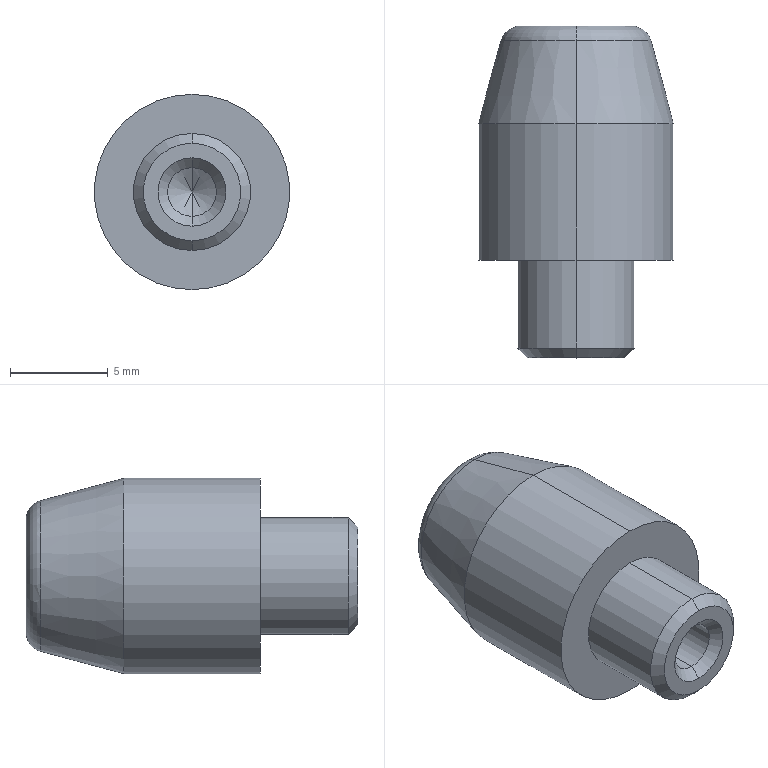Component | SolidWorks | MA060.03.03-02-1 | 1 solid | 19 faces | box 10 x 17 x 10 mm | volume 944 mm3 | cone 8 | cylinder 6 | plane 3 | torus 2 | commonest cylinder face diameters 2.5 x2 6 x2 10 x2 | material 45#
build123d program:
from build123d import *

# Parameters (mm, degrees)
M3_TAPPED_HOLE1_D     = 2.5
M3_TAPPED_HOLE1_DEPTH = 7.5
M3_TAPPED_HOLE1_TIP   = 0.7511
CHAMFER1_SIZE         = 0.5
CHAMFER2_SIZE         = 5
CHAMFER2_SIZE2        = 1.34
FILLET1_R             = 1


with BuildPart() as part:
    # Sketch1 → Revolve1 (revolve)
    with BuildSketch(Plane.XY, mode=Mode.PRIVATE) as revolve1_sk:
        Polygon((0, 0), (0, 17), (5, 17), (5, 5), (3, 5), (3, 0), align=None)
    revolve(revolve1_sk.sketch.rotate(Axis((0, 0, 0), (0, 1, 0)), 90), axis=Axis((0, 0, 0), (0, 1, 0)))

    # M3 Tapped Hole1
    with Locations(Plane(origin=(0, 0, 0), x_dir=(0, 0, -1), z_dir=(0, -1, 0))):
        with Locations((0, 0)):
            Hole(M3_TAPPED_HOLE1_D / 2, depth=M3_TAPPED_HOLE1_DEPTH)
            with Locations((0, 0, -(M3_TAPPED_HOLE1_DEPTH + M3_TAPPED_HOLE1_TIP / 2))):  # 118° drill point
                Cone(0, M3_TAPPED_HOLE1_D / 2, M3_TAPPED_HOLE1_TIP, mode=Mode.SUBTRACT)

    # Chamfer1
    chamfer1_edges = [part.edges().sort_by_distance(p)[0] for p in [
        (0, 0, -1.25),
        (0, 0, 3),
    ]]
    chamfer(chamfer1_edges, length=CHAMFER1_SIZE)

    # Chamfer2
    chamfer2_edges = [part.edges().sort_by_distance(p)[0] for p in [
        (0, 17, 5),
    ]]
    chamfer2_side = [part.faces().sort_by_distance(p)[0] for p in [
        (0, 11, 5),
    ]]
    chamfer(chamfer2_edges, length=CHAMFER2_SIZE, length2=CHAMFER2_SIZE2, reference=chamfer2_side[0])

    # Fillet1
    fillet1_edges = [part.edges().sort_by_distance(p)[0] for p in [
        (0, 17, 3.66),
    ]]
    fillet(fillet1_edges, radius=FILLET1_R)


solid = part.part

# Placed as in the assembly
solid = solid.moved(Location((-41, 73.053, 0), (0, 0, 0)))
STEP:
#1=CARTESIAN_POINT('',(-1.614,3.516,-0.1519));
#2=VERTEX_POINT('',#1);
#3=CARTESIAN_POINT('',(-1.614,3.516,0.1519));
#4=VERTEX_POINT('',#3);
#5=CARTESIAN_POINT('',(-1.614,3.516,-0.));
#6=DIRECTION('',(0.,-1.,0.));
#7=DIRECTION('',(0.,0.,1.));
#8=AXIS2_PLACEMENT_3D('',#5,#6,#7);
#9=CIRCLE('',#8,0.1519);
#10=EDGE_CURVE('',#2,#4,#9,.T.);
#11=ORIENTED_EDGE('',*,*,#10,.F.);
#12=CARTESIAN_POINT('',(-1.614,3.545,-0.1139));
#13=VERTEX_POINT('',#12);
#14=CARTESIAN_POINT('',(-1.614,3.506,-0.1139));
#15=DIRECTION('',(1.,0.,0.));
#16=DIRECTION('',(0.,0.,-1.));
#17=AXIS2_PLACEMENT_3D('',#14,#15,#16);
#18=CIRCLE('',#17,0.03937);
#19=EDGE_CURVE('',#2,#13,#18,.T.);
#20=ORIENTED_EDGE('',*,*,#19,.T.);
#21=CARTESIAN_POINT('',(-1.614,3.545,0.1139));
#22=VERTEX_POINT('',#21);
#23=CARTESIAN_POINT('',(-1.614,3.545,-0.));
#24=DIRECTION('',(0.,1.,0.));
#25=DIRECTION('',(0.,0.,1.));
#26=AXIS2_PLACEMENT_3D('',#23,#24,#25);
#27=CIRCLE('',#26,0.1139);
#28=EDGE_CURVE('',#22,#13,#27,.T.);
#29=ORIENTED_EDGE('',*,*,#28,.F.);
#30=CARTESIAN_POINT('',(-1.614,3.506,0.1139));
#31=DIRECTION('',(-1.,0.,0.));
#32=DIRECTION('',(0.,0.,1.));
#33=AXIS2_PLACEMENT_3D('',#30,#31,#32);
#34=CIRCLE('',#33,0.03937);
#35=EDGE_CURVE('',#4,#22,#34,.T.);
#36=ORIENTED_EDGE('',*,*,#35,.F.);
#37=EDGE_LOOP('',(#11,#20,#29,#36));
#38=FACE_OUTER_BOUND('',#37,.T.);
#39=CARTESIAN_POINT('',(-1.614,3.506,-0.));
#40=DIRECTION('',(0.,1.,0.));
#41=DIRECTION('',(0.,0.,1.));
#42=AXIS2_PLACEMENT_3D('',#39,#40,#41);
#43=TOROIDAL_SURFACE('',#42,0.1139,0.03937);
#44=ADVANCED_FACE('',(#38),#43,.T.);
#45=ORIENTED_EDGE('',*,*,#10,.T.);
#46=CARTESIAN_POINT('',(-1.614,3.349,0.1969));
#47=VERTEX_POINT('',#46);
#48=CARTESIAN_POINT('',(-1.614,3.349,0.1969));
#49=DIRECTION('',(0.,-0.9659,0.2588));
#50=VECTOR('',#49,39.37);
#51=LINE('',#48,#50);
#52=EDGE_CURVE('',#4,#47,#51,.T.);
#53=ORIENTED_EDGE('',*,*,#52,.T.);
#54=CARTESIAN_POINT('',(-1.614,3.349,-0.1969));
#55=VERTEX_POINT('',#54);
#56=CARTESIAN_POINT('',(-1.614,3.349,-0.));
#57=DIRECTION('',(0.,-1.,0.));
#58=DIRECTION('',(0.,0.,1.));
#59=AXIS2_PLACEMENT_3D('',#56,#57,#58);
#60=CIRCLE('',#59,0.1969);
#61=EDGE_CURVE('',#55,#47,#60,.T.);
#62=ORIENTED_EDGE('',*,*,#61,.F.);
#63=CARTESIAN_POINT('',(-1.614,3.349,-0.1969));
#64=DIRECTION('',(0.,-0.9659,-0.2588));
#65=VECTOR('',#64,39.37);
#66=LINE('',#63,#65);
#67=EDGE_CURVE('',#2,#55,#66,.T.);
#68=ORIENTED_EDGE('',*,*,#67,.F.);
#69=EDGE_LOOP('',(#45,#53,#62,#68));
#70=FACE_OUTER_BOUND('',#69,.T.);
#71=CARTESIAN_POINT('',(-1.614,3.349,-0.));
#72=DIRECTION('',(0.,-1.,0.));
#73=DIRECTION('',(0.,0.,-1.));
#74=AXIS2_PLACEMENT_3D('',#71,#72,#73);
#75=CONICAL_SURFACE('',#74,0.1969,0.2618);
#76=ADVANCED_FACE('',(#70),#75,.T.);
#77=CARTESIAN_POINT('',(-1.614,2.896,0.04921));
#78=VERTEX_POINT('',#77);
#79=CARTESIAN_POINT('',(-1.614,2.896,-0.04921));
#80=VERTEX_POINT('',#79);
#81=CARTESIAN_POINT('',(-1.614,2.896,-0.));
#82=DIRECTION('',(0.,-1.,0.));
#83=DIRECTION('',(0.,0.,-1.));
#84=AXIS2_PLACEMENT_3D('',#81,#82,#83);
#85=CIRCLE('',#84,0.04921);
#86=EDGE_CURVE('',#78,#80,#85,.T.);
#87=ORIENTED_EDGE('',*,*,#86,.F.);
#88=CARTESIAN_POINT('',(-1.614,2.876,0.0689));
#89=VERTEX_POINT('',#88);
#90=CARTESIAN_POINT('',(-1.614,2.896,0.04921));
#91=DIRECTION('',(0.,-0.7071,0.7071));
#92=VECTOR('',#91,39.37);
#93=LINE('',#90,#92);
#94=EDGE_CURVE('',#78,#89,#93,.T.);
#95=ORIENTED_EDGE('',*,*,#94,.T.);
#96=CARTESIAN_POINT('',(-1.614,2.876,-0.0689));
#97=VERTEX_POINT('',#96);
#98=CARTESIAN_POINT('',(-1.614,2.876,-0.));
#99=DIRECTION('',(0.,1.,0.));
#100=DIRECTION('',(0.,0.,-1.));
#101=AXIS2_PLACEMENT_3D('',#98,#99,#100);
#102=CIRCLE('',#101,0.0689);
#103=EDGE_CURVE('',#97,#89,#102,.T.);
#104=ORIENTED_EDGE('',*,*,#103,.F.);
#105=CARTESIAN_POINT('',(-1.614,2.896,-0.04921));
#106=DIRECTION('',(0.,-0.7071,-0.7071));
#107=VECTOR('',#106,39.37);
#108=LINE('',#105,#107);
#109=EDGE_CURVE('',#80,#97,#108,.T.);
#110=ORIENTED_EDGE('',*,*,#109,.F.);
#111=EDGE_LOOP('',(#87,#95,#104,#110));
#112=FACE_OUTER_BOUND('',#111,.T.);
#113=CARTESIAN_POINT('',(-1.614,2.896,-0.));
#114=DIRECTION('',(0.,-1.,0.));
#115=DIRECTION('',(0.,0.,-1.));
#116=AXIS2_PLACEMENT_3D('',#113,#114,#115);
#117=CONICAL_SURFACE('',#116,0.04921,0.7854);
#118=ADVANCED_FACE('',(#112),#117,.F.);
#119=CARTESIAN_POINT('',(-1.614,2.876,-0.09843));
#120=VERTEX_POINT('',#119);
#121=CARTESIAN_POINT('',(-1.614,2.876,0.09843));
#122=VERTEX_POINT('',#121);
#123=CARTESIAN_POINT('',(-1.614,2.876,-0.));
#124=DIRECTION('',(0.,-1.,0.));
#125=DIRECTION('',(0.,0.,-1.));
#126=AXIS2_PLACEMENT_3D('',#123,#124,#125);
#127=CIRCLE('',#126,0.09843);
#128=EDGE_CURVE('',#120,#122,#127,.T.);
#129=ORIENTED_EDGE('',*,*,#128,.F.);
#130=CARTESIAN_POINT('',(-1.614,2.896,-0.1181));
#131=VERTEX_POINT('',#130);
#132=CARTESIAN_POINT('',(-1.614,2.876,-0.09843));
#133=DIRECTION('',(0.,0.7071,-0.7071));
#134=VECTOR('',#133,39.37);
#135=LINE('',#132,#134);
#136=EDGE_CURVE('',#120,#131,#135,.T.);
#137=ORIENTED_EDGE('',*,*,#136,.T.);
#138=CARTESIAN_POINT('',(-1.614,2.896,0.1181));
#139=VERTEX_POINT('',#138);
#140=CARTESIAN_POINT('',(-1.614,2.896,-0.));
#141=DIRECTION('',(0.,1.,0.));
#142=DIRECTION('',(0.,0.,-1.));
#143=AXIS2_PLACEMENT_3D('',#140,#141,#142);
#144=CIRCLE('',#143,0.1181);
#145=EDGE_CURVE('',#139,#131,#144,.T.);
#146=ORIENTED_EDGE('',*,*,#145,.F.);
#147=CARTESIAN_POINT('',(-1.614,2.876,0.09843));
#148=DIRECTION('',(0.,0.7071,0.7071));
#149=VECTOR('',#148,39.37);
#150=LINE('',#147,#149);
#151=EDGE_CURVE('',#122,#139,#150,.T.);
#152=ORIENTED_EDGE('',*,*,#151,.F.);
#153=EDGE_LOOP('',(#129,#137,#146,#152));
#154=FACE_OUTER_BOUND('',#153,.T.);
#155=CARTESIAN_POINT('',(-1.614,2.876,-0.));
#156=DIRECTION('',(0.,1.,0.));
#157=DIRECTION('',(0.,0.,1.));
#158=AXIS2_PLACEMENT_3D('',#155,#156,#157);
#159=CONICAL_SURFACE('',#158,0.09843,0.7854);
#160=ADVANCED_FACE('',(#154),#159,.T.);
#161=CARTESIAN_POINT('',(-1.614,3.171,0.04921));
#162=VERTEX_POINT('',#161);
#163=CARTESIAN_POINT('',(-1.614,3.171,-0.04921));
#164=VERTEX_POINT('',#163);
#165=CARTESIAN_POINT('',(-1.614,3.171,-0.));
#166=DIRECTION('',(0.,-1.,0.));
#167=DIRECTION('',(0.,0.,-1.));
#168=AXIS2_PLACEMENT_3D('',#165,#166,#167);
#169=CIRCLE('',#168,0.04921);
#170=EDGE_CURVE('',#162,#164,#169,.T.);
#171=ORIENTED_EDGE('',*,*,#170,.F.);
#172=CARTESIAN_POINT('',(-1.614,2.876,0.04921));
#173=DIRECTION('',(0.,-1.,0.));
#174=VECTOR('',#173,39.37);
#175=LINE('',#172,#174);
#176=EDGE_CURVE('',#162,#78,#175,.T.);
#177=ORIENTED_EDGE('',*,*,#176,.T.);
#178=ORIENTED_EDGE('',*,*,#86,.T.);
#179=CARTESIAN_POINT('',(-1.614,2.876,-0.04921));
#180=DIRECTION('',(0.,-1.,0.));
#181=VECTOR('',#180,39.37);
#182=LINE('',#179,#181);
#183=EDGE_CURVE('',#164,#80,#182,.T.);
#184=ORIENTED_EDGE('',*,*,#183,.F.);
#185=EDGE_LOOP('',(#171,#177,#178,#184));
#186=FACE_OUTER_BOUND('',#185,.T.);
#187=CARTESIAN_POINT('',(-1.614,2.876,-0.));
#188=DIRECTION('',(0.,-1.,0.));
#189=DIRECTION('',(0.,0.,-1.));
#190=AXIS2_PLACEMENT_3D('',#187,#188,#189);
#191=CYLINDRICAL_SURFACE('',#190,0.04921);
#192=ADVANCED_FACE('',(#186),#191,.F.);
#193=CARTESIAN_POINT('',(-1.614,3.201,-0.));
#194=VERTEX_POINT('',#193);
#195=CARTESIAN_POINT('',(-1.614,3.171,-0.04921));
#196=DIRECTION('',(0.,-0.515,-0.8572));
#197=VECTOR('',#196,39.37);
#198=LINE('',#195,#197);
#199=EDGE_CURVE('',#194,#164,#198,.T.);
#200=ORIENTED_EDGE('',*,*,#199,.F.);
#201=CARTESIAN_POINT('',(-1.614,3.171,0.04921));
#202=DIRECTION('',(0.,-0.515,0.8572));
#203=VECTOR('',#202,39.37);
#204=LINE('',#201,#203);
#205=EDGE_CURVE('',#194,#162,#204,.T.);
#206=ORIENTED_EDGE('',*,*,#205,.T.);
#207=ORIENTED_EDGE('',*,*,#170,.T.);
#208=EDGE_LOOP('',(#200,#206,#207));
#209=FACE_OUTER_BOUND('',#208,.T.);
#210=CARTESIAN_POINT('',(-1.614,3.171,-0.));
#211=DIRECTION('',(0.,-1.,0.));
#212=DIRECTION('',(0.,0.,-1.));
#213=AXIS2_PLACEMENT_3D('',#210,#211,#212);
#214=CONICAL_SURFACE('',#213,0.04921,1.03);
#215=ADVANCED_FACE('',(#209),#214,.F.);
#216=CARTESIAN_POINT('',(-1.614,3.073,-0.1181));
#217=VERTEX_POINT('',#216);
#218=CARTESIAN_POINT('',(-1.614,3.073,0.1181));
#219=VERTEX_POINT('',#218);
#220=CARTESIAN_POINT('',(-1.614,3.073,-0.));
#221=DIRECTION('',(0.,-1.,0.));
#222=DIRECTION('',(0.,0.,-1.));
#223=AXIS2_PLACEMENT_3D('',#220,#221,#222);
#224=CIRCLE('',#223,0.1181);
#225=EDGE_CURVE('',#217,#219,#224,.T.);
#226=ORIENTED_EDGE('',*,*,#225,.T.);
#227=CARTESIAN_POINT('',(-1.614,2.876,0.1181));
#228=DIRECTION('',(0.,-1.,0.));
#229=VECTOR('',#228,39.37);
#230=LINE('',#227,#229);
#231=EDGE_CURVE('',#219,#139,#230,.T.);
#232=ORIENTED_EDGE('',*,*,#231,.T.);
#233=ORIENTED_EDGE('',*,*,#145,.T.);
#234=CARTESIAN_POINT('',(-1.614,2.876,-0.1181));
#235=DIRECTION('',(0.,-1.,0.));
#236=VECTOR('',#235,39.37);
#237=LINE('',#234,#236);
#238=EDGE_CURVE('',#217,#131,#237,.T.);
#239=ORIENTED_EDGE('',*,*,#238,.F.);
#240=EDGE_LOOP('',(#226,#232,#233,#239));
#241=FACE_OUTER_BOUND('',#240,.T.);
#242=CARTESIAN_POINT('',(-1.614,2.876,-0.));
#243=DIRECTION('',(0.,-1.,0.));
#244=DIRECTION('',(0.,0.,-1.));
#245=AXIS2_PLACEMENT_3D('',#242,#243,#244);
#246=CYLINDRICAL_SURFACE('',#245,0.1181);
#247=ADVANCED_FACE('',(#241),#246,.T.);
#248=ORIENTED_EDGE('',*,*,#61,.T.);
#249=CARTESIAN_POINT('',(-1.614,3.073,0.1969));
#250=VERTEX_POINT('',#249);
#251=CARTESIAN_POINT('',(-1.614,2.876,0.1969));
#252=DIRECTION('',(0.,-1.,0.));
#253=VECTOR('',#252,39.37);
#254=LINE('',#251,#253);
#255=EDGE_CURVE('',#47,#250,#254,.T.);
#256=ORIENTED_EDGE('',*,*,#255,.T.);
#257=CARTESIAN_POINT('',(-1.614,3.073,-0.1969));
#258=VERTEX_POINT('',#257);
#259=CARTESIAN_POINT('',(-1.614,3.073,-0.));
#260=DIRECTION('',(0.,-1.,0.));
#261=DIRECTION('',(0.,0.,-1.));
#262=AXIS2_PLACEMENT_3D('',#259,#260,#261);
#263=CIRCLE('',#262,0.1969);
#264=EDGE_CURVE('',#258,#250,#263,.T.);
#265=ORIENTED_EDGE('',*,*,#264,.F.);
#266=CARTESIAN_POINT('',(-1.614,2.876,-0.1969));
#267=DIRECTION('',(0.,-1.,0.));
#268=VECTOR('',#267,39.37);
#269=LINE('',#266,#268);
#270=EDGE_CURVE('',#55,#258,#269,.T.);
#271=ORIENTED_EDGE('',*,*,#270,.F.);
#272=EDGE_LOOP('',(#248,#256,#265,#271));
#273=FACE_OUTER_BOUND('',#272,.T.);
#274=CARTESIAN_POINT('',(-1.614,2.876,-0.));
#275=DIRECTION('',(0.,-1.,0.));
#276=DIRECTION('',(0.,0.,-1.));
#277=AXIS2_PLACEMENT_3D('',#274,#275,#276);
#278=CYLINDRICAL_SURFACE('',#277,0.1969);
#279=ADVANCED_FACE('',(#273),#278,.T.);
#280=CARTESIAN_POINT('',(-1.614,2.876,-0.));
#281=DIRECTION('',(0.,-1.,0.));
#282=DIRECTION('',(0.,0.,-1.));
#283=AXIS2_PLACEMENT_3D('',#280,#281,#282);
#284=CIRCLE('',#283,0.09843);
#285=EDGE_CURVE('',#122,#120,#284,.T.);
#286=ORIENTED_EDGE('',*,*,#285,.T.);
#287=ORIENTED_EDGE('',*,*,#128,.T.);
#288=EDGE_LOOP('',(#286,#287));
#289=FACE_OUTER_BOUND('',#288,.T.);
#290=ORIENTED_EDGE('',*,*,#103,.T.);
#291=CARTESIAN_POINT('',(-1.614,2.876,-0.));
#292=DIRECTION('',(0.,1.,0.));
#293=DIRECTION('',(0.,0.,-1.));
#294=AXIS2_PLACEMENT_3D('',#291,#292,#293);
#295=CIRCLE('',#294,0.0689);
#296=EDGE_CURVE('',#89,#97,#295,.T.);
#297=ORIENTED_EDGE('',*,*,#296,.T.);
#298=EDGE_LOOP('',(#290,#297));
#299=FACE_BOUND('',#298,.T.);
#300=CARTESIAN_POINT('',(-1.496,2.876,-0.));
#301=DIRECTION('',(0.,-1.,0.));
#302=DIRECTION('',(0.,0.,-1.));
#303=AXIS2_PLACEMENT_3D('',#300,#301,#302);
#304=PLANE('',#303);
#305=ADVANCED_FACE('',(#289,#299),#304,.T.);
#306=ORIENTED_EDGE('',*,*,#28,.T.);
#307=CARTESIAN_POINT('',(-1.614,3.545,-0.));
#308=DIRECTION('',(0.,1.,0.));
#309=DIRECTION('',(0.,0.,1.));
#310=AXIS2_PLACEMENT_3D('',#307,#308,#309);
#311=CIRCLE('',#310,0.1139);
#312=EDGE_CURVE('',#13,#22,#311,.T.);
#313=ORIENTED_EDGE('',*,*,#312,.T.);
#314=EDGE_LOOP('',(#306,#313));
#315=FACE_OUTER_BOUND('',#314,.T.);
#316=CARTESIAN_POINT('',(-1.614,3.545,-0.));
#317=DIRECTION('',(0.,1.,0.));
#318=DIRECTION('',(0.,0.,1.));
#319=AXIS2_PLACEMENT_3D('',#316,#317,#318);
#320=PLANE('',#319);
#321=ADVANCED_FACE('',(#315),#320,.T.);
#322=ORIENTED_EDGE('',*,*,#255,.F.);
#323=CARTESIAN_POINT('',(-1.614,3.349,-0.));
#324=DIRECTION('',(0.,-1.,0.));
#325=DIRECTION('',(0.,0.,1.));
#326=AXIS2_PLACEMENT_3D('',#323,#324,#325);
#327=CIRCLE('',#326,0.1969);
#328=EDGE_CURVE('',#47,#55,#327,.T.);
#329=ORIENTED_EDGE('',*,*,#328,.T.);
#330=ORIENTED_EDGE('',*,*,#270,.T.);
#331=CARTESIAN_POINT('',(-1.614,3.073,-0.));
#332=DIRECTION('',(0.,-1.,0.));
#333=DIRECTION('',(0.,0.,-1.));
#334=AXIS2_PLACEMENT_3D('',#331,#332,#333);
#335=CIRCLE('',#334,0.1969);
#336=EDGE_CURVE('',#250,#258,#335,.T.);
#337=ORIENTED_EDGE('',*,*,#336,.F.);
#338=EDGE_LOOP('',(#322,#329,#330,#337));
#339=FACE_OUTER_BOUND('',#338,.T.);
#340=CARTESIAN_POINT('',(-1.614,2.876,-0.));
#341=DIRECTION('',(0.,-1.,0.));
#342=DIRECTION('',(0.,0.,-1.));
#343=AXIS2_PLACEMENT_3D('',#340,#341,#342);
#344=CYLINDRICAL_SURFACE('',#343,0.1969);
#345=ADVANCED_FACE('',(#339),#344,.T.);
#346=ORIENTED_EDGE('',*,*,#264,.T.);
#347=ORIENTED_EDGE('',*,*,#336,.T.);
#348=EDGE_LOOP('',(#346,#347));
#349=FACE_OUTER_BOUND('',#348,.T.);
#350=ORIENTED_EDGE('',*,*,#225,.F.);
#351=CARTESIAN_POINT('',(-1.614,3.073,-0.));
#352=DIRECTION('',(0.,-1.,0.));
#353=DIRECTION('',(0.,0.,-1.));
#354=AXIS2_PLACEMENT_3D('',#351,#352,#353);
#355=CIRCLE('',#354,0.1181);
#356=EDGE_CURVE('',#219,#217,#355,.T.);
#357=ORIENTED_EDGE('',*,*,#356,.F.);
#358=EDGE_LOOP('',(#350,#357));
#359=FACE_BOUND('',#358,.T.);
#360=CARTESIAN_POINT('',(-1.417,3.073,-0.));
#361=DIRECTION('',(0.,-1.,0.));
#362=DIRECTION('',(0.,0.,-1.));
#363=AXIS2_PLACEMENT_3D('',#360,#361,#362);
#364=PLANE('',#363);
#365=ADVANCED_FACE('',(#349,#359),#364,.T.);
#366=ORIENTED_EDGE('',*,*,#231,.F.);
#367=ORIENTED_EDGE('',*,*,#356,.T.);
#368=ORIENTED_EDGE('',*,*,#238,.T.);
#369=CARTESIAN_POINT('',(-1.614,2.896,-0.));
#370=DIRECTION('',(0.,1.,0.));
#371=DIRECTION('',(0.,0.,-1.));
#372=AXIS2_PLACEMENT_3D('',#369,#370,#371);
#373=CIRCLE('',#372,0.1181);
#374=EDGE_CURVE('',#131,#139,#373,.T.);
#375=ORIENTED_EDGE('',*,*,#374,.T.);
#376=EDGE_LOOP('',(#366,#367,#368,#375));
#377=FACE_OUTER_BOUND('',#376,.T.);
#378=CARTESIAN_POINT('',(-1.614,2.876,-0.));
#379=DIRECTION('',(0.,-1.,0.));
#380=DIRECTION('',(0.,0.,-1.));
#381=AXIS2_PLACEMENT_3D('',#378,#379,#380);
#382=CYLINDRICAL_SURFACE('',#381,0.1181);
#383=ADVANCED_FACE('',(#377),#382,.T.);
#384=ORIENTED_EDGE('',*,*,#205,.F.);
#385=ORIENTED_EDGE('',*,*,#199,.T.);
#386=CARTESIAN_POINT('',(-1.614,3.171,-0.));
#387=DIRECTION('',(0.,-1.,0.));
#388=DIRECTION('',(0.,0.,-1.));
#389=AXIS2_PLACEMENT_3D('',#386,#387,#388);
#390=CIRCLE('',#389,0.04921);
#391=EDGE_CURVE('',#164,#162,#390,.T.);
#392=ORIENTED_EDGE('',*,*,#391,.T.);
#393=EDGE_LOOP('',(#384,#385,#392));
#394=FACE_OUTER_BOUND('',#393,.T.);
#395=CARTESIAN_POINT('',(-1.614,3.171,-0.));
#396=DIRECTION('',(0.,-1.,0.));
#397=DIRECTION('',(0.,0.,-1.));
#398=AXIS2_PLACEMENT_3D('',#395,#396,#397);
#399=CONICAL_SURFACE('',#398,0.04921,1.03);
#400=ADVANCED_FACE('',(#394),#399,.F.);
#401=ORIENTED_EDGE('',*,*,#176,.F.);
#402=ORIENTED_EDGE('',*,*,#391,.F.);
#403=ORIENTED_EDGE('',*,*,#183,.T.);
#404=CARTESIAN_POINT('',(-1.614,2.896,-0.));
#405=DIRECTION('',(0.,-1.,0.));
#406=DIRECTION('',(0.,0.,-1.));
#407=AXIS2_PLACEMENT_3D('',#404,#405,#406);
#408=CIRCLE('',#407,0.04921);
#409=EDGE_CURVE('',#80,#78,#408,.T.);
#410=ORIENTED_EDGE('',*,*,#409,.T.);
#411=EDGE_LOOP('',(#401,#402,#403,#410));
#412=FACE_OUTER_BOUND('',#411,.T.);
#413=CARTESIAN_POINT('',(-1.614,2.876,-0.));
#414=DIRECTION('',(0.,-1.,0.));
#415=DIRECTION('',(0.,0.,-1.));
#416=AXIS2_PLACEMENT_3D('',#413,#414,#415);
#417=CYLINDRICAL_SURFACE('',#416,0.04921);
#418=ADVANCED_FACE('',(#412),#417,.F.);
#419=ORIENTED_EDGE('',*,*,#136,.F.);
#420=ORIENTED_EDGE('',*,*,#285,.F.);
#421=ORIENTED_EDGE('',*,*,#151,.T.);
#422=ORIENTED_EDGE('',*,*,#374,.F.);
#423=EDGE_LOOP('',(#419,#420,#421,#422));
#424=FACE_OUTER_BOUND('',#423,.T.);
#425=CARTESIAN_POINT('',(-1.614,2.876,-0.));
#426=DIRECTION('',(0.,1.,0.));
#427=DIRECTION('',(0.,0.,1.));
#428=AXIS2_PLACEMENT_3D('',#425,#426,#427);
#429=CONICAL_SURFACE('',#428,0.09843,0.7854);
#430=ADVANCED_FACE('',(#424),#429,.T.);
#431=ORIENTED_EDGE('',*,*,#94,.F.);
#432=ORIENTED_EDGE('',*,*,#409,.F.);
#433=ORIENTED_EDGE('',*,*,#109,.T.);
#434=ORIENTED_EDGE('',*,*,#296,.F.);
#435=EDGE_LOOP('',(#431,#432,#433,#434));
#436=FACE_OUTER_BOUND('',#435,.T.);
#437=CARTESIAN_POINT('',(-1.614,2.896,-0.));
#438=DIRECTION('',(0.,-1.,0.));
#439=DIRECTION('',(0.,0.,-1.));
#440=AXIS2_PLACEMENT_3D('',#437,#438,#439);
#441=CONICAL_SURFACE('',#440,0.04921,0.7854);
#442=ADVANCED_FACE('',(#436),#441,.F.);
#443=ORIENTED_EDGE('',*,*,#52,.F.);
#444=CARTESIAN_POINT('',(-1.614,3.516,-0.));
#445=DIRECTION('',(0.,-1.,0.));
#446=DIRECTION('',(0.,0.,1.));
#447=AXIS2_PLACEMENT_3D('',#444,#445,#446);
#448=CIRCLE('',#447,0.1519);
#449=EDGE_CURVE('',#4,#2,#448,.T.);
#450=ORIENTED_EDGE('',*,*,#449,.T.);
#451=ORIENTED_EDGE('',*,*,#67,.T.);
#452=ORIENTED_EDGE('',*,*,#328,.F.);
#453=EDGE_LOOP('',(#443,#450,#451,#452));
#454=FACE_OUTER_BOUND('',#453,.T.);
#455=CARTESIAN_POINT('',(-1.614,3.349,-0.));
#456=DIRECTION('',(0.,-1.,0.));
#457=DIRECTION('',(0.,0.,-1.));
#458=AXIS2_PLACEMENT_3D('',#455,#456,#457);
#459=CONICAL_SURFACE('',#458,0.1969,0.2618);
#460=ADVANCED_FACE('',(#454),#459,.T.);
#461=ORIENTED_EDGE('',*,*,#19,.F.);
#462=ORIENTED_EDGE('',*,*,#449,.F.);
#463=ORIENTED_EDGE('',*,*,#35,.T.);
#464=ORIENTED_EDGE('',*,*,#312,.F.);
#465=EDGE_LOOP('',(#461,#462,#463,#464));
#466=FACE_OUTER_BOUND('',#465,.T.);
#467=CARTESIAN_POINT('',(-1.614,3.506,-0.));
#468=DIRECTION('',(0.,1.,0.));
#469=DIRECTION('',(0.,0.,1.));
#470=AXIS2_PLACEMENT_3D('',#467,#468,#469);
#471=TOROIDAL_SURFACE('',#470,0.1139,0.03937);
#472=ADVANCED_FACE('',(#466),#471,.T.);
#473=CLOSED_SHELL('',(#44,#76,#118,#160,#192,#215,#247,#279,#305,#321,#345,#365,#383,#400,#418,#430,#442,#460,#472));
#474=MANIFOLD_SOLID_BREP('',#473);
#475=CARTESIAN_POINT('',(0.,0.,0.));
#476=DIRECTION('',(0.,0.,1.));
#477=DIRECTION('',(1.,0.,0.));
#478=AXIS2_PLACEMENT_3D('',#475,#476,#477);
#479=(LENGTH_UNIT()NAMED_UNIT(*)SI_UNIT($,.METRE.));
#480=LENGTH_MEASURE_WITH_UNIT(LENGTH_MEASURE(0.0254),#479);
#481=DIMENSIONAL_EXPONENTS(1.,0.,0.,0.,0.,0.,0.);
#482=(CONVERSION_BASED_UNIT('',#480)LENGTH_UNIT()NAMED_UNIT(#481));
#483=UNCERTAINTY_MEASURE_WITH_UNIT(LENGTH_MEASURE(0.00001),#482,'','');
#484=(NAMED_UNIT(*)PLANE_ANGLE_UNIT()SI_UNIT($,.RADIAN.));
#485=(NAMED_UNIT(*)SI_UNIT($,.STERADIAN.)SOLID_ANGLE_UNIT());
#486=(GEOMETRIC_REPRESENTATION_CONTEXT(3)GLOBAL_UNCERTAINTY_ASSIGNED_CONTEXT((#483))GLOBAL_UNIT_ASSIGNED_CONTEXT((#482,#484,#485))REPRESENTATION_CONTEXT('',''));
#487=ADVANCED_BREP_SHAPE_REPRESENTATION('',(#474,#478),#486);
#488=COLOUR_RGB('',0.7922,0.8196,0.9333);
#489=FILL_AREA_STYLE_COLOUR('',#488);
#490=FILL_AREA_STYLE('',(#489));
#491=SURFACE_STYLE_FILL_AREA(#490);
#492=SURFACE_SIDE_STYLE('',(#491));
#493=SURFACE_STYLE_USAGE(.BOTH.,#492);
#494=PRESENTATION_STYLE_ASSIGNMENT((#493));
#495=STYLED_ITEM('',(#494),#474);
#496=(LENGTH_UNIT()NAMED_UNIT(*)SI_UNIT($,.METRE.));
#497=LENGTH_MEASURE_WITH_UNIT(LENGTH_MEASURE(0.0254),#496);
#498=DIMENSIONAL_EXPONENTS(1.,0.,0.,0.,0.,0.,0.);
#499=(CONVERSION_BASED_UNIT('',#497)LENGTH_UNIT()NAMED_UNIT(#498));
#500=UNCERTAINTY_MEASURE_WITH_UNIT(LENGTH_MEASURE(0.00001),#499,'','');
#501=(NAMED_UNIT(*)PLANE_ANGLE_UNIT()SI_UNIT($,.RADIAN.));
#502=(NAMED_UNIT(*)SI_UNIT($,.STERADIAN.)SOLID_ANGLE_UNIT());
#503=(GEOMETRIC_REPRESENTATION_CONTEXT(3)GLOBAL_UNCERTAINTY_ASSIGNED_CONTEXT((#500))GLOBAL_UNIT_ASSIGNED_CONTEXT((#499,#501,#502))REPRESENTATION_CONTEXT('',''));
#504=MECHANICAL_DESIGN_GEOMETRIC_PRESENTATION_REPRESENTATION('',(#495),#503);
#505=PRESENTATION_LAYER_ASSIGNMENT('','',(#495));